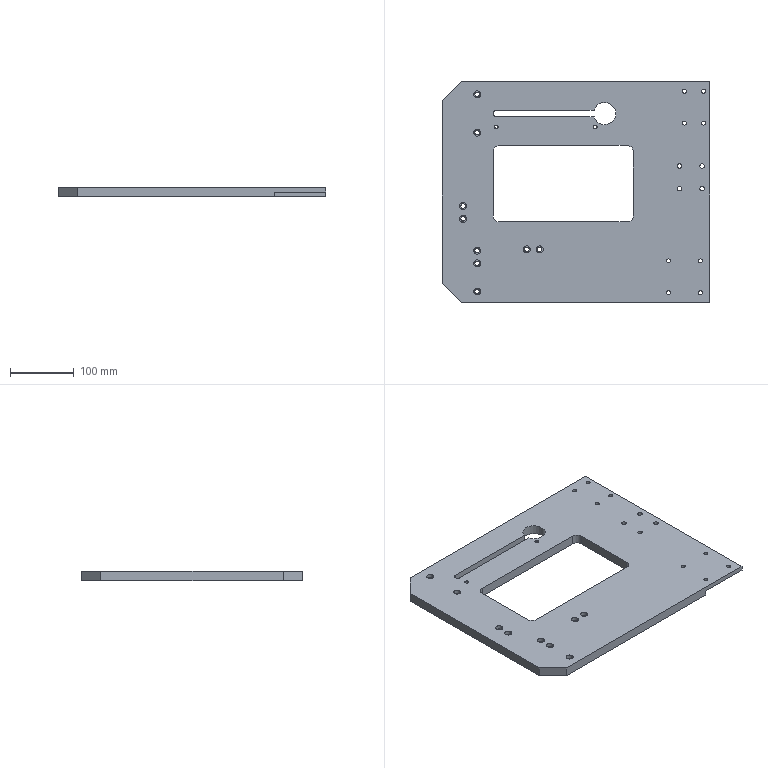Component | SolidWorks | LargeSidePlate(1)-1 | 1 solid | 103 faces | box 420 x 346 x 15 mm | volume 1642209 mm3 | cylinder 70 | plane 29 | cone 4 | commonest cylinder face diameters 7 x26 11 x18 6.2 x16 5 x4 20 x4 10.2 x1 35 x1
build123d program:
from build123d import *

# Parameters (mm, degrees)
SKETCH1_W                                            = 420
SKETCH1_H                                            = 346
BOSS_EXTRUDE1_DEPTH                                  = 15
SKETCH2_W                                            = 220
SKETCH2_H                                            = 120
CUT_EXTRUDE1_DEPTH                                   = 455.482
CUT_EXTRUDE2_DEPTH                                   = 455.482
SKETCH4_W                                            = 50
SKETCH4_H                                            = 80
CUT_EXTRUDE3_DEPTH                                   = 7.5
SKETCH5_W                                            = 80
SKETCH5_H                                            = 80
CUT_EXTRUDE4_DEPTH                                   = 7.5
SKETCH6_W                                            = 17.5
SKETCH6_H                                            = 15
F_7_0_7_DIAMETER_HOLE1_D                             = 7
F_6_2_6_2_DIAMETER_HOLE1_D                           = 6.2
F_6_2_6_2_DIAMETER_HOLE1_DEPTH                       = 15
F_5_0_5_DIAMETER_HOLE1_D                             = 5
CYLINDRICAL_COUNTERSUNK_HOLE1_FOR_M6_HEX_D           = 7
CYLINDRICAL_COUNTERSUNK_HOLE1_FOR_M6_HEX_CBORE_D     = 11
CYLINDRICAL_COUNTERSUNK_HOLE1_FOR_M6_HEX_CBORE_DEPTH = 6
CHAMFER1_SIZE                                        = 0.525
CHAMFER2_SIZE                                        = 30
FILLET1_R                                            = 10


with BuildPart() as part:
    # Sketch1 → Boss-Extrude1 (new body)
    with BuildSketch(Plane(origin=(0, 0, -7.5), x_dir=(-1, 0, 0), z_dir=(0, 0, -1))):
        with Locations((210, 0)):
            Rectangle(SKETCH1_W, SKETCH1_H)
    extrude(amount=-BOSS_EXTRUDE1_DEPTH)

    # Sketch2 → Cut-Extrude1 (cut, through all)
    with BuildSketch(Plane(origin=(0, 0, -7.5), x_dir=(-1, 0, 0), z_dir=(0, 0, -1))):
        with Locations((230, 13)):
            Rectangle(SKETCH2_W, SKETCH2_H)
    extrude(amount=-CUT_EXTRUDE1_DEPTH, mode=Mode.SUBTRACT)

    # Sketch3 → Cut-Extrude2 (cut, through all)
    with BuildSketch(Plane.XY.offset(7.5)):
        with BuildLine():
            Line((-335, 117.9), (-181.74, 117.9))
            ThreePointArc((-181.74, 117.9), (-182.5, 123), (-181.74, 128.1))
            Line((-181.74, 128.1), (-335, 128.1))
            ThreePointArc((-335, 128.1), (-340.1, 123), (-335, 117.9))
        make_face()
    extrude(amount=-CUT_EXTRUDE2_DEPTH, mode=Mode.SUBTRACT)

    # Sketch4 → Cut-Extrude3 (cut)
    with BuildSketch(Plane(origin=(0, 0, -7.5), x_dir=(-1, 0, 0), z_dir=(0, 0, -1))):
        with Locations((25, 133)):
            Rectangle(SKETCH4_W, SKETCH4_H)
    extrude(amount=-CUT_EXTRUDE3_DEPTH, mode=Mode.SUBTRACT)

    # Sketch5 → Cut-Extrude4 (cut)
    with BuildSketch(Plane(origin=(0, 0, -7.5), x_dir=(-1, 0, 0), z_dir=(0, 0, -1))):
        with Locations((40, -133)):
            Rectangle(SKETCH5_W, SKETCH5_H)
    extrude(amount=-CUT_EXTRUDE4_DEPTH, mode=Mode.SUBTRACT)

    # Sketch6 → Cut-Revolve1 (revolve, cut)
    with BuildSketch(Plane.XZ.offset(-123)):
        with Locations((-156.25, 0)):
            Rectangle(SKETCH6_W, SKETCH6_H)
    revolve(axis=Axis((-165, 123, 7.5), (0, 0, -1)), mode=Mode.SUBTRACT)

    # 7.0 _7_ Diameter Hole1 (through all)
    with Locations(Plane.XY.offset(7.5)):
        with Locations((-12.322, 5.322), (-47.678, 40.678), (-12.322, 40.678), (-47.678, 5.322)):
            Hole(F_7_0_7_DIAMETER_HOLE1_D / 2)

    # 6.2 _6.2_ Diameter Hole1
    with Locations(Plane.XY.offset(7.5)):
        with Locations((-65, -158), (-65, -108), (-40, 108), (-40, 158), (-10, 158), (-10, 108), (-15, -108), (-15, -158)):
            Hole(F_6_2_6_2_DIAMETER_HOLE1_D / 2, depth=F_6_2_6_2_DIAMETER_HOLE1_DEPTH)

    # 5.0 _5_ Diameter Hole1 (through all)
    with Locations(Plane.XY.offset(7.5)):
        with Locations((-335, 102), (-180, 102)):
            Hole(F_5_0_5_DIAMETER_HOLE1_D / 2)

    # Cylindrical Countersunk Hole1 for M6 Hex (through all)
    with Locations(Plane.XY.offset(7.5)):
        with Locations((-365, 153), (-365, 93), (-387, -22), (-387, -42), (-365, -92), (-365, -112), (-365, -156), (-287, -90), (-267, -90)):
            CounterBoreHole(CYLINDRICAL_COUNTERSUNK_HOLE1_FOR_M6_HEX_D / 2, CYLINDRICAL_COUNTERSUNK_HOLE1_FOR_M6_HEX_CBORE_D / 2, CYLINDRICAL_COUNTERSUNK_HOLE1_FOR_M6_HEX_CBORE_DEPTH)

    # Chamfer1
    chamfer1_edges = [part.edges().sort_by_distance(p)[0] for p in [
        (-177.5, 102, 7.5),
        (-332.5, 102, 7.5),
    ]]
    chamfer(chamfer1_edges, length=CHAMFER1_SIZE)

    # Chamfer2
    chamfer2_edges = [part.edges().sort_by_distance(p)[0] for p in [
        (-420, -173, 0),
        (-420, 173, 0),
    ]]
    chamfer(chamfer2_edges, length=CHAMFER2_SIZE)

    # Fillet1
    fillet1_edges = [part.edges().sort_by_distance(p)[0] for p in [
        (-120, 73, 0),
        (-340, 73, 0),
        (-340, -47, 0),
        (-120, -47, 0),
    ]]
    fillet(fillet1_edges, radius=FILLET1_R)


solid = part.part

# Placed as in the assembly
solid = solid.moved(Location((0, 438, 270), (0, 0, 0)))